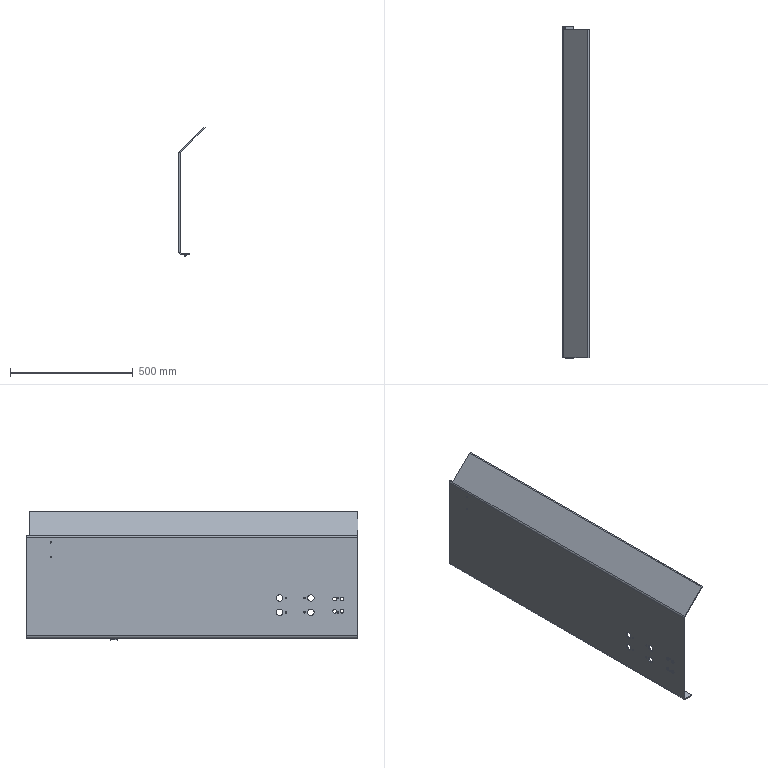Component | SolidWorks | 004FrameSheet-MetalA-1 | 3 solids | 60 faces | box 107.07 x 1350 x 523 mm | volume 3980317 mm3 | cylinder 41 | plane 19 | commonest cylinder face diameters 5 x10 15 x8 6.5 x8 26 x8 4 x2 10 x2 20 x2 8 x1 | material Plain Carbon Steel
build123d program:
from build123d import *

# Parameters (mm, degrees)
SKETCH2_W                  = 410
SKETCH2_H                  = 515
BOSS_EXTRUDE1_DEPTH        = 1350
FILLET1_R                  = 10
CHAMFER1_SIZE              = 100
FILLET3_R                  = 10
SHELL1_T                   = -5
CUT_EXTRUDE1_REACH         = 1461.366
SKETCH3_W                  = 320
SKETCH3_H                  = 1561.085
SKETCH7_R                  = 13
SKETCH7_R_2                = 3.25
CUT_EXTRUDE5_DEPTH         = 5
SKETCH8_R                  = 7.5
CUT_EXTRUDE6_DEPTH         = 5
M6_TAPPED_HOLE1_AT_2_COUNT = 2
M6_TAPPED_HOLE1_AT_2_PITCH = 60
SKETCH13_R                 = 20
CUT_EXTRUDE7_DEPTH         = 5
M6_TAPPED_HOLE3_AT_2_COUNT = 2
M6_TAPPED_HOLE3_AT_2_PITCH = 60
CUT_EXTRUDE9_DEPTH         = 1390.544
SKETCH18_W                 = 400
SKETCH18_H                 = 15
CUT_EXTRUDE11_DEPTH        = 1390.544
CUT_EXTRUDE10_DEPTH        = 1390.544
CUT_EXTRUDE10_DEPTH_BACK   = 1390.544
SKETCH16_W                 = 275.063
SKETCH16_H                 = 1482.264
BOSS_EXTRUDE3_DEPTH        = 1335
BOSS_EXTRUDE4_START        = -345
SKETCH20_R                 = 2
BOSS_EXTRUDE4_DEPTH        = 25


with BuildPart() as part:
    # Sketch2 → Boss-Extrude1 (new body)
    with BuildSketch(Plane(origin=(0, 0, 0), x_dir=(1, 0, 0), z_dir=(0, 1, 0))):
        Rectangle(SKETCH2_W, SKETCH2_H)
    extrude(amount=BOSS_EXTRUDE1_DEPTH)

    # Fillet1
    fillet1_edges = [part.edges().sort_by_distance(p)[0] for p in [
        (-205, 675, -257.5),
        (205, 675, -257.5),
    ]]
    fillet(fillet1_edges, radius=FILLET1_R)

    # Chamfer1
    chamfer1_edges = [part.edges().sort_by_distance(p)[0] for p in [
        (205, 675, 257.5),
        (-205, 675, 257.5),
    ]]
    chamfer(chamfer1_edges, length=CHAMFER1_SIZE)

    # Fillet3
    fillet3_edges = [part.edges().sort_by_distance(p)[0] for p in [
        (205, 675, 157.5),
        (-205, 675, 157.5),
    ]]
    fillet(fillet3_edges, radius=FILLET3_R)

    # Shell1
    shell1_openings = [part.faces().sort_by_distance(p)[0] for p in [
        (0, 1350, -11.096),
        (0, 0, -11.096),
        (0, 675, 257.5),
    ]]
    offset(amount=SHELL1_T, openings=shell1_openings, kind=Kind.INTERSECTION)

    # Sketch3 → Cut-Extrude1 (cut, up to next)
    with BuildSketch(Plane(origin=(0, 0, -257.5), x_dir=(-1, 0, 0), z_dir=(0, 0, -1)), mode=Mode.PRIVATE) as cut_extrude1_sk1:
        with Locations((0, 708.71)):
            Rectangle(SKETCH3_W, SKETCH3_H)
    cut_extrude1_tool1 = extrude(cut_extrude1_sk1.sketch, amount=-CUT_EXTRUDE1_REACH, mode=Mode.PRIVATE) & part.part
    add(cut_extrude1_tool1.solids().sort_by_distance((0, 708.71, -257.5))[0], mode=Mode.SUBTRACT)


with BuildPart() as cut_extrude1_piece_1:
    # of the separate pieces the step leaves, piece 1, a body of its own (cut_extrude1_pieces)
    add(part.part.solids().sort_by_distance((195, 0, -257.5))[0])

    # Sketch13 → Cut-Extrude7 (cut)
    with BuildSketch(Plane(origin=(205, 0, 0), x_dir=(0, 0, -1), z_dir=(1, 0, 0))):
        with Locations((102.5, 950)):
            Circle(SKETCH13_R)
    extrude(amount=-CUT_EXTRUDE7_DEPTH, mode=Mode.SUBTRACT)


with BuildPart() as cut_extrude1_piece_2:
    # of the separate pieces the step leaves, piece 2, a body of its own (cut_extrude1_pieces)
    add(part.part.solids().sort_by_distance((-202.071, 0, 160.429))[0])

    # Sketch7 → Cut-Extrude5 (cut)
    with BuildSketch(Plane.ZY.offset(205)):
        with Locations((-151.5, 191.5)):
            Circle(SKETCH7_R)
        with Locations((-151.5, 318.5)):
            Circle(SKETCH7_R)
        with Locations((-151.5, 293)):
            Circle(SKETCH7_R_2)
        with Locations((-151.5, 217)):
            Circle(SKETCH7_R_2)
        with Locations((-93.5, 191.5)):
            Circle(SKETCH7_R)
        with Locations((-93.5, 318.5)):
            Circle(SKETCH7_R)
        with Locations((-93.5, 217)):
            Circle(SKETCH7_R_2)
        with Locations((-93.5, 293)):
            Circle(SKETCH7_R_2)
    extrude(amount=-CUT_EXTRUDE5_DEPTH, mode=Mode.SUBTRACT)

    # Sketch8 → Cut-Extrude6 (cut)
    with BuildSketch(Plane.ZY.offset(205)):
        with Locations((-147.5, 95)):
            Circle(SKETCH8_R)
        with Locations((-97.5, 95)):
            Circle(SKETCH8_R)
        with Locations((-147.5, 65)):
            Circle(SKETCH8_R)
        with Locations((-97.5, 65)):
            Circle(SKETCH8_R)
    extrude(amount=-CUT_EXTRUDE6_DEPTH, mode=Mode.SUBTRACT)

    # Sketch9 → M6 Tapped Hole1 (revolve, cut)
    with BuildSketch(Plane(origin=(-205, 80, -92.5), x_dir=(0, 0, 1), z_dir=(0, 1, 0))):
        Polygon((0, 0), (0, 16.502), (2.5, 15), (2.5, 0), align=None)
    m6_tapped_hole1 = revolve(axis=Axis((-211.35, 80, -92.5), (1, 0, 0)), mode=Mode.SUBTRACT)

    # M6 Tapped Hole1 at 2: M6 Tapped Hole1 ×2
    with Locations(*[(0, 0, -i * M6_TAPPED_HOLE1_AT_2_PITCH) for i in range(1, M6_TAPPED_HOLE1_AT_2_COUNT)]):
        add(m6_tapped_hole1, mode=Mode.SUBTRACT)

    # Sketch14 → M6 Tapped Hole3 (revolve, cut)
    with BuildSketch(Plane(origin=(-205, 1250, 72.5), x_dir=(0, 0, 1), z_dir=(0, 1, 0))):
        Polygon((0, 0), (0, 16.502), (2.5, 15), (2.5, 0), align=None)
    m6_tapped_hole3 = revolve(axis=Axis((-211.35, 1250, 72.5), (1, 0, 0)), mode=Mode.SUBTRACT)

    # M6 Tapped Hole3 at 2: M6 Tapped Hole3 ×2
    with Locations(*[(0, 0, i * M6_TAPPED_HOLE3_AT_2_PITCH) for i in range(1, M6_TAPPED_HOLE3_AT_2_COUNT)]):
        add(m6_tapped_hole3, mode=Mode.SUBTRACT)


with BuildPart() as cut_extrude9_tool:
    # Sketch17 → Cut-Extrude9 (new, through all)
    with BuildSketch(Plane(origin=(0, 1350, 0), x_dir=(1, 0, 0), z_dir=(0, 1, 0))):
        Polygon((-105, -257.5), (0, -152.5), (105, -257.5), align=None)
    extrude(amount=-CUT_EXTRUDE9_DEPTH)


with BuildPart() as cut_extrude1_piece_1_1:
    add(cut_extrude1_piece_1.part)

    # Cut-Extrude9: cut by cut_extrude9_tool
    add(cut_extrude9_tool.part, mode=Mode.SUBTRACT)


with BuildPart() as cut_extrude1_piece_2_1:
    add(cut_extrude1_piece_2.part)

    # Cut-Extrude9: cut by cut_extrude9_tool
    add(cut_extrude9_tool.part, mode=Mode.SUBTRACT)


with BuildPart() as cut_extrude11_tool:
    # Sketch18 → Cut-Extrude11 (new, through all)
    with BuildSketch(Plane.XY):
        with Locations((0, 1342.5)):
            Rectangle(SKETCH18_W, SKETCH18_H)
    extrude(amount=CUT_EXTRUDE11_DEPTH)


with BuildPart() as cut_extrude1_piece_1_2:
    add(cut_extrude1_piece_1_1.part)

    # Cut-Extrude11: cut by cut_extrude11_tool
    add(cut_extrude11_tool.part, mode=Mode.SUBTRACT)

    # Sketch16 → Cut-Extrude10 (cut, two sides: drawn at the far end of the back side and taken through both)
    with BuildSketch(Plane.XY.offset(-CUT_EXTRUDE10_DEPTH_BACK)):
        with Locations((137.531, 741.132)):
            Rectangle(SKETCH16_W, SKETCH16_H)
    extrude(amount=CUT_EXTRUDE10_DEPTH + CUT_EXTRUDE10_DEPTH_BACK, mode=Mode.SUBTRACT)


with BuildPart() as cut_extrude1_piece_2_2:
    add(cut_extrude1_piece_2_1.part)

    # Cut-Extrude11: cut by cut_extrude11_tool
    add(cut_extrude11_tool.part, mode=Mode.SUBTRACT)


with BuildPart() as body_2:
    # Sketch19 → Boss-Extrude3 (new, through all)
    with BuildSketch(Plane(origin=(0, 1335, 0), x_dir=(1, 0, 0), z_dir=(0, 1, 0))):
        Polygon((-105, -257.5), (-97.929, -257.5), (-101.464, -253.964), align=None)
    extrude(amount=-BOSS_EXTRUDE3_DEPTH)


with BuildPart() as body_3:
    # Sketch20 → Boss-Extrude4 (new body)
    with BuildSketch(Plane(origin=(0, 1350, 0), x_dir=(1, 0, 0), z_dir=(0, 1, 0)).offset(BOSS_EXTRUDE4_START)):
        with BuildLine():
            Line((-172.675, 257.5), (-185.325, 257.5))
            ThreePointArc((-185.325, 257.5), (-183.363, 258.45), (-182.892, 260.577))
            ThreePointArc((-182.892, 260.577), (-179, 265.5), (-175.108, 260.577))
            ThreePointArc((-175.108, 260.577), (-174.637, 258.45), (-172.675, 257.5))
        make_face()
        with Locations(Location((-179, 261.5, 0), (0, 0, 270))):
            Circle(SKETCH20_R, mode=Mode.SUBTRACT)
    extrude(amount=-BOSS_EXTRUDE4_DEPTH)


solid = Compound([cut_extrude1_piece_2_2.part, body_2.part, body_3.part])

# Placed as in the assembly
solid = solid.moved(Location((160, 37, -262.5), (0, 0, 0)))